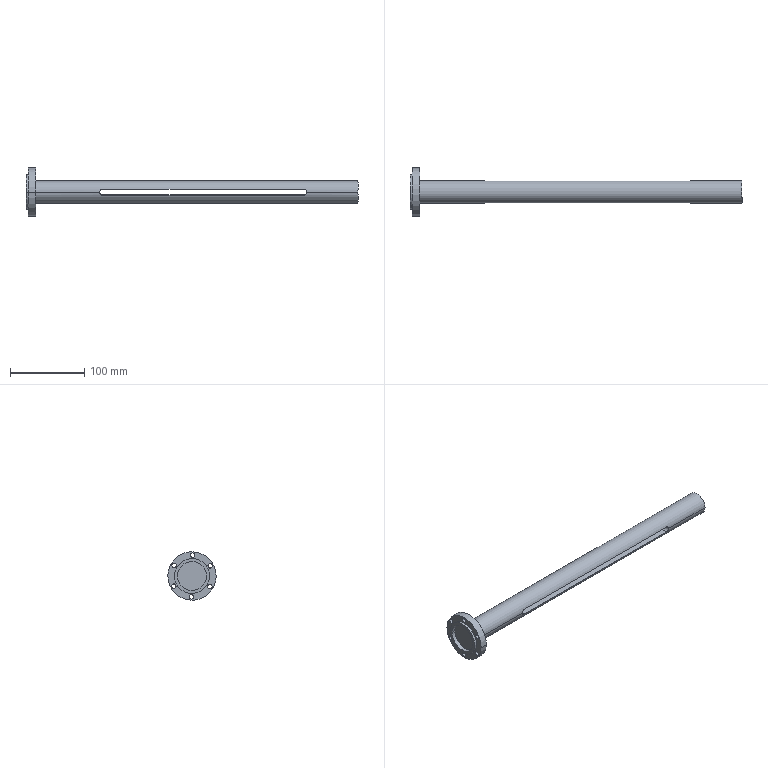Component | SolidWorks | TailstockAxis-1 | 1 solid | 33 faces | box 446 x 65 x 65 mm | volume 269234 mm3 | cylinder 25 | plane 8 | commonest cylinder face diameters 6 x12 8 x3 12 x2 30 x2 65 x2 47 x2 39 x2
build123d program:
from build123d import *

# Parameters (mm, degrees)
SKETCH2_R                             = 3
CUT_EXTRUDE1_DEPTH                    = 20
CUT_EXTRUDE2_DEPTH                    = 20
M12_PISTON_ROD_THREADED_HOLE_SKETCH_R = 6
M12_PISTON_ROD_THREADED_HOLE_DEPTH    = 18


with BuildPart() as part:
    # Sketch1 → Revolve1 (revolve)
    with BuildSketch(Plane.XY, mode=Mode.PRIVATE) as revolve1_sk:
        Polygon((0, 19.5), (0, 23.5), (3, 23.5), (3, 32.5), (13, 32.5), (13, 15), (446, 15), (446, 0), (5, 0), (5, 19.5), align=None)
    revolve(revolve1_sk.sketch.rotate(Axis((-33.776, 0, 0), (1, 0, 0)), 90), axis=Axis((-33.776, 0, 0), (1, 0, 0)))

    # Sketch2 → Cut-Extrude1 (cut)
    with BuildSketch(Plane.ZY.offset(-3)):
        with Locations((0, 28)):
            Circle(SKETCH2_R)
        with Locations((24.249, 14)):
            Circle(SKETCH2_R)
        with Locations((24.249, -14)):
            Circle(SKETCH2_R)
        with Locations((0, -28)):
            Circle(SKETCH2_R)
        with Locations((-24.249, -14)):
            Circle(SKETCH2_R)
        with Locations((-24.249, 14)):
            Circle(SKETCH2_R)
    extrude(amount=-CUT_EXTRUDE1_DEPTH, mode=Mode.SUBTRACT)

    # Sketch3 → Cut-Extrude2 (cut, symmetric)
    with BuildSketch(Plane.XY):
        with BuildLine():
            Line((103, 4), (373, 4))
            ThreePointArc((373, 4), (377, 0), (373, -4))
            Line((373, -4), (103, -4))
            ThreePointArc((103, -4), (99, 0), (103, 4))
        make_face()
    extrude(amount=CUT_EXTRUDE2_DEPTH, both=True, mode=Mode.SUBTRACT)

    # M12 Piston Rod Threaded Hole Sketch → M12 Piston Rod Threaded Hole (cut)
    with BuildSketch(Plane(origin=(446, 0, 0), x_dir=(0, 0, -1), z_dir=(1, 0, 0))):
        Circle(M12_PISTON_ROD_THREADED_HOLE_SKETCH_R)
    extrude(amount=-M12_PISTON_ROD_THREADED_HOLE_DEPTH, mode=Mode.SUBTRACT)


solid = part.part

# Placed as in the assembly
solid = solid.moved(Location((465.936, 1299.706, 687.116), (-89, 0, 0)))